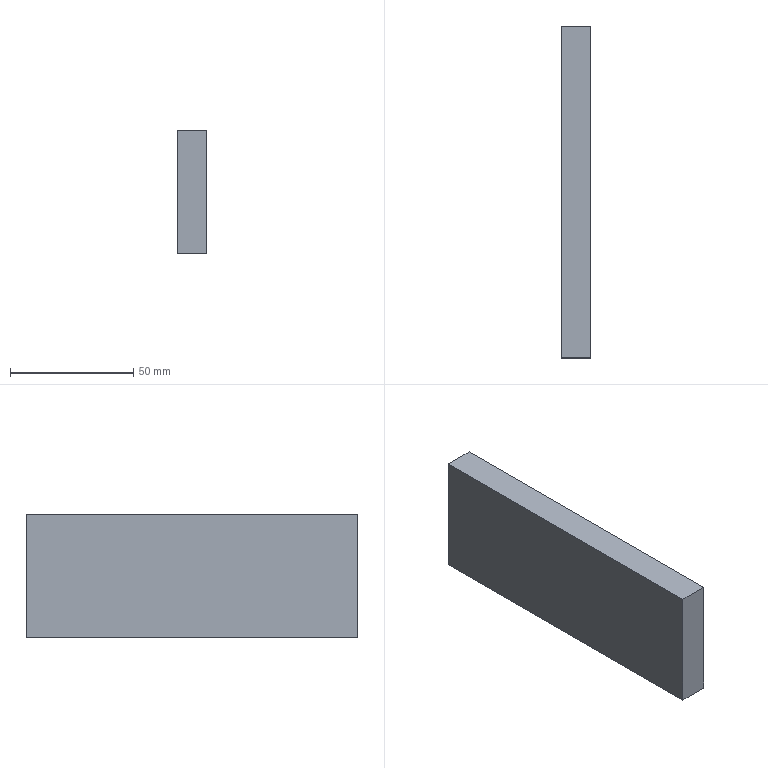Component | SolidWorks | HZ022-A001-E005-1 | 1 solid | 6 faces | box 12 x 134.5 x 50 mm | volume 80700 mm3 | plane 6 | material AL6061
build123d program:
from build123d import *

# Parameters (mm, degrees)
SKETCH1_W           = 134.5
SKETCH1_H           = 50
BOSS_EXTRUDE1_DEPTH = 12


with BuildPart() as part:
    # Sketch1 → Boss-Extrude1 (new body)
    with BuildSketch(Plane(origin=(0, 0, 0), x_dir=(1, 0, 0), z_dir=(0, 1, 0))):
        Rectangle(SKETCH1_W, SKETCH1_H)
    extrude(amount=BOSS_EXTRUDE1_DEPTH)


solid = part.part

# Placed as in the assembly
solid = solid.moved(Location((-282.556, 81.902, 924.5), (0, 0, 90)))
STEP:
#1=COLOUR_RGB('',0.7922,0.8196,0.9333);
#2=FILL_AREA_STYLE_COLOUR('',#1);
#3=FILL_AREA_STYLE('',(#2));
#4=SURFACE_STYLE_FILL_AREA(#3);
#5=SURFACE_SIDE_STYLE('',(#4));
#6=SURFACE_STYLE_USAGE(.BOTH.,#5);
#7=PRESENTATION_STYLE_ASSIGNMENT((#6));
#8=CARTESIAN_POINT('',(-11.597,0.5769,37.382));
#9=VERTEX_POINT('',#8);
#10=CARTESIAN_POINT('',(-11.597,0.5769,35.413));
#11=VERTEX_POINT('',#10);
#12=CARTESIAN_POINT('',(-11.597,0.5769,35.413));
#13=DIRECTION('',(-0.,0.,-1.));
#14=VECTOR('',#13,39.37);
#15=LINE('',#12,#14);
#16=EDGE_CURVE('',#9,#11,#15,.T.);
#17=ORIENTED_EDGE('',*,*,#16,.T.);
#18=CARTESIAN_POINT('',(-11.124,0.5769,35.413));
#19=VERTEX_POINT('',#18);
#20=CARTESIAN_POINT('',(-11.124,0.5769,35.413));
#21=DIRECTION('',(-1.,-0.,0.));
#22=VECTOR('',#21,39.37);
#23=LINE('',#20,#22);
#24=EDGE_CURVE('',#19,#11,#23,.T.);
#25=ORIENTED_EDGE('',*,*,#24,.F.);
#26=CARTESIAN_POINT('',(-11.124,0.5769,37.382));
#27=VERTEX_POINT('',#26);
#28=CARTESIAN_POINT('',(-11.124,0.5769,35.413));
#29=DIRECTION('',(-0.,0.,-1.));
#30=VECTOR('',#29,39.37);
#31=LINE('',#28,#30);
#32=EDGE_CURVE('',#27,#19,#31,.T.);
#33=ORIENTED_EDGE('',*,*,#32,.F.);
#34=CARTESIAN_POINT('',(-11.124,0.5769,37.382));
#35=DIRECTION('',(-1.,-0.,0.));
#36=VECTOR('',#35,39.37);
#37=LINE('',#34,#36);
#38=EDGE_CURVE('',#27,#9,#37,.T.);
#39=ORIENTED_EDGE('',*,*,#38,.T.);
#40=EDGE_LOOP('',(#17,#25,#33,#39));
#41=FACE_OUTER_BOUND('',#40,.T.);
#42=CARTESIAN_POINT('',(-11.124,0.5769,35.413));
#43=DIRECTION('',(-0.,1.,0.));
#44=DIRECTION('',(0.,-0.,1.));
#45=AXIS2_PLACEMENT_3D('',#42,#43,#44);
#46=PLANE('',#45);
#47=ADVANCED_FACE('',(#41),#46,.F.);
#48=CARTESIAN_POINT('',(-11.597,5.872,35.413));
#49=VERTEX_POINT('',#48);
#50=CARTESIAN_POINT('',(-11.597,5.872,35.413));
#51=DIRECTION('',(-0.,1.,0.));
#52=VECTOR('',#51,39.37);
#53=LINE('',#50,#52);
#54=EDGE_CURVE('',#11,#49,#53,.T.);
#55=ORIENTED_EDGE('',*,*,#54,.T.);
#56=CARTESIAN_POINT('',(-11.124,5.872,35.413));
#57=VERTEX_POINT('',#56);
#58=CARTESIAN_POINT('',(-11.124,5.872,35.413));
#59=DIRECTION('',(-1.,-0.,0.));
#60=VECTOR('',#59,39.37);
#61=LINE('',#58,#60);
#62=EDGE_CURVE('',#57,#49,#61,.T.);
#63=ORIENTED_EDGE('',*,*,#62,.F.);
#64=CARTESIAN_POINT('',(-11.124,5.872,35.413));
#65=DIRECTION('',(-0.,1.,0.));
#66=VECTOR('',#65,39.37);
#67=LINE('',#64,#66);
#68=EDGE_CURVE('',#19,#57,#67,.T.);
#69=ORIENTED_EDGE('',*,*,#68,.F.);
#70=ORIENTED_EDGE('',*,*,#24,.T.);
#71=EDGE_LOOP('',(#55,#63,#69,#70));
#72=FACE_OUTER_BOUND('',#71,.T.);
#73=CARTESIAN_POINT('',(-11.124,5.872,35.413));
#74=DIRECTION('',(0.,-0.,1.));
#75=DIRECTION('',(0.,-1.,-0.));
#76=AXIS2_PLACEMENT_3D('',#73,#74,#75);
#77=PLANE('',#76);
#78=ADVANCED_FACE('',(#72),#77,.F.);
#79=CARTESIAN_POINT('',(-11.597,5.872,37.382));
#80=VERTEX_POINT('',#79);
#81=CARTESIAN_POINT('',(-11.597,5.872,35.413));
#82=DIRECTION('',(0.,-0.,1.));
#83=VECTOR('',#82,39.37);
#84=LINE('',#81,#83);
#85=EDGE_CURVE('',#49,#80,#84,.T.);
#86=ORIENTED_EDGE('',*,*,#85,.T.);
#87=CARTESIAN_POINT('',(-11.124,5.872,37.382));
#88=VERTEX_POINT('',#87);
#89=CARTESIAN_POINT('',(-11.124,5.872,37.382));
#90=DIRECTION('',(-1.,-0.,0.));
#91=VECTOR('',#90,39.37);
#92=LINE('',#89,#91);
#93=EDGE_CURVE('',#88,#80,#92,.T.);
#94=ORIENTED_EDGE('',*,*,#93,.F.);
#95=CARTESIAN_POINT('',(-11.124,5.872,35.413));
#96=DIRECTION('',(0.,-0.,1.));
#97=VECTOR('',#96,39.37);
#98=LINE('',#95,#97);
#99=EDGE_CURVE('',#57,#88,#98,.T.);
#100=ORIENTED_EDGE('',*,*,#99,.F.);
#101=ORIENTED_EDGE('',*,*,#62,.T.);
#102=EDGE_LOOP('',(#86,#94,#100,#101));
#103=FACE_OUTER_BOUND('',#102,.T.);
#104=CARTESIAN_POINT('',(-11.124,5.872,35.413));
#105=DIRECTION('',(0.,-1.,-0.));
#106=DIRECTION('',(-0.,0.,-1.));
#107=AXIS2_PLACEMENT_3D('',#104,#105,#106);
#108=PLANE('',#107);
#109=ADVANCED_FACE('',(#103),#108,.F.);
#110=CARTESIAN_POINT('',(-11.597,5.872,37.382));
#111=DIRECTION('',(0.,-1.,-0.));
#112=VECTOR('',#111,39.37);
#113=LINE('',#110,#112);
#114=EDGE_CURVE('',#80,#9,#113,.T.);
#115=ORIENTED_EDGE('',*,*,#114,.T.);
#116=ORIENTED_EDGE('',*,*,#38,.F.);
#117=CARTESIAN_POINT('',(-11.124,5.872,37.382));
#118=DIRECTION('',(0.,-1.,-0.));
#119=VECTOR('',#118,39.37);
#120=LINE('',#117,#119);
#121=EDGE_CURVE('',#88,#27,#120,.T.);
#122=ORIENTED_EDGE('',*,*,#121,.F.);
#123=ORIENTED_EDGE('',*,*,#93,.T.);
#124=EDGE_LOOP('',(#115,#116,#122,#123));
#125=FACE_OUTER_BOUND('',#124,.T.);
#126=CARTESIAN_POINT('',(-11.124,5.872,37.382));
#127=DIRECTION('',(-0.,0.,-1.));
#128=DIRECTION('',(-0.,1.,0.));
#129=AXIS2_PLACEMENT_3D('',#126,#127,#128);
#130=PLANE('',#129);
#131=ADVANCED_FACE('',(#125),#130,.F.);
#132=ORIENTED_EDGE('',*,*,#32,.T.);
#133=ORIENTED_EDGE('',*,*,#68,.T.);
#134=ORIENTED_EDGE('',*,*,#99,.T.);
#135=ORIENTED_EDGE('',*,*,#121,.T.);
#136=EDGE_LOOP('',(#132,#133,#134,#135));
#137=FACE_OUTER_BOUND('',#136,.T.);
#138=CARTESIAN_POINT('',(-11.124,3.224,36.398));
#139=DIRECTION('',(1.,0.,-0.));
#140=DIRECTION('',(0.,-0.,1.));
#141=AXIS2_PLACEMENT_3D('',#138,#139,#140);
#142=PLANE('',#141);
#143=ADVANCED_FACE('',(#137),#142,.T.);
#144=ORIENTED_EDGE('',*,*,#16,.F.);
#145=ORIENTED_EDGE('',*,*,#114,.F.);
#146=ORIENTED_EDGE('',*,*,#85,.F.);
#147=ORIENTED_EDGE('',*,*,#54,.F.);
#148=EDGE_LOOP('',(#144,#145,#146,#147));
#149=FACE_OUTER_BOUND('',#148,.T.);
#150=CARTESIAN_POINT('',(-11.597,3.224,36.398));
#151=DIRECTION('',(1.,0.,-0.));
#152=DIRECTION('',(0.,-0.,1.));
#153=AXIS2_PLACEMENT_3D('',#150,#151,#152);
#154=PLANE('',#153);
#155=ADVANCED_FACE('',(#149),#154,.F.);
#156=CLOSED_SHELL('',(#47,#78,#109,#131,#143,#155));
#157=MANIFOLD_SOLID_BREP('',#156);
#158=STYLED_ITEM('',(#7),#157);
#159=PRESENTATION_LAYER_ASSIGNMENT('','',(#158));
#160=CARTESIAN_POINT('',(0.,0.,0.));
#161=DIRECTION('',(0.,0.,1.));
#162=DIRECTION('',(1.,0.,0.));
#163=AXIS2_PLACEMENT_3D('',#160,#161,#162);
#164=(LENGTH_UNIT()NAMED_UNIT(*)SI_UNIT($,.METRE.));
#165=LENGTH_MEASURE_WITH_UNIT(LENGTH_MEASURE(0.0254),#164);
#166=DIMENSIONAL_EXPONENTS(1.,0.,0.,0.,0.,0.,0.);
#167=(CONVERSION_BASED_UNIT('',#165)LENGTH_UNIT()NAMED_UNIT(#166));
#168=UNCERTAINTY_MEASURE_WITH_UNIT(LENGTH_MEASURE(0.00001),#167,'','');
#169=(NAMED_UNIT(*)PLANE_ANGLE_UNIT()SI_UNIT($,.RADIAN.));
#170=(NAMED_UNIT(*)SI_UNIT($,.STERADIAN.)SOLID_ANGLE_UNIT());
#171=(GEOMETRIC_REPRESENTATION_CONTEXT(3)GLOBAL_UNCERTAINTY_ASSIGNED_CONTEXT((#168))GLOBAL_UNIT_ASSIGNED_CONTEXT((#167,#169,#170))REPRESENTATION_CONTEXT('',''));
#172=ADVANCED_BREP_SHAPE_REPRESENTATION('',(#157,#163),#171);
#173=(LENGTH_UNIT()NAMED_UNIT(*)SI_UNIT($,.METRE.));
#174=LENGTH_MEASURE_WITH_UNIT(LENGTH_MEASURE(0.0254),#173);
#175=DIMENSIONAL_EXPONENTS(1.,0.,0.,0.,0.,0.,0.);
#176=(CONVERSION_BASED_UNIT('',#174)LENGTH_UNIT()NAMED_UNIT(#175));
#177=UNCERTAINTY_MEASURE_WITH_UNIT(LENGTH_MEASURE(0.00001),#176,'','');
#178=(NAMED_UNIT(*)PLANE_ANGLE_UNIT()SI_UNIT($,.RADIAN.));
#179=(NAMED_UNIT(*)SI_UNIT($,.STERADIAN.)SOLID_ANGLE_UNIT());
#180=(GEOMETRIC_REPRESENTATION_CONTEXT(3)GLOBAL_UNCERTAINTY_ASSIGNED_CONTEXT((#177))GLOBAL_UNIT_ASSIGNED_CONTEXT((#176,#178,#179))REPRESENTATION_CONTEXT('',''));
#181=MECHANICAL_DESIGN_GEOMETRIC_PRESENTATION_REPRESENTATION('',(#158),#180);